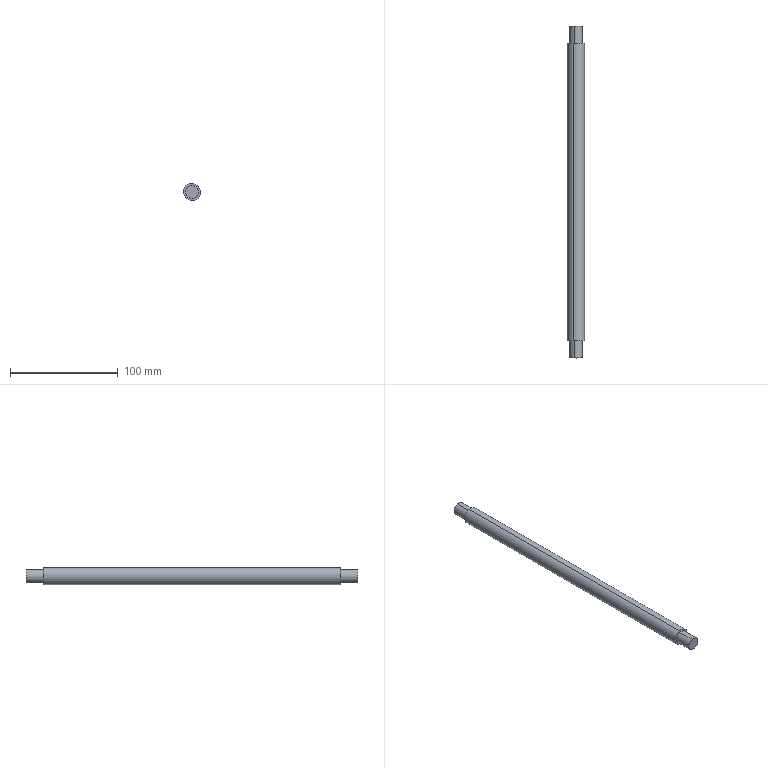Component | SolidWorks | AdjustmentRod-2 | 1 solid | 10 faces | box 16 x 308 x 16 mm | volume 59112 mm3 | cylinder 6 | plane 4 | commonest cylinder face diameters 12 x4 16 x2
build123d program:
from build123d import *


with BuildPart() as part:
    # Sketch1 → Revolve1 (revolve)
    with BuildSketch(Plane.XY, mode=Mode.PRIVATE) as revolve1_sk:
        Polygon((6, 154), (6, 138), (8, 138), (8, -138), (6, -138), (6, -154), (0, -154), (0, 154), align=None)
    revolve(revolve1_sk.sketch.rotate(Axis((0, 0, 0), (0, 1, 0)), 90), axis=Axis((0, 0, 0), (0, 1, 0)))


solid = part.part

# Placed as in the assembly
solid = solid.moved(Location((-155, 0, 0), (0, 0, 0)))
STEP:
#1=COLOUR_RGB('',0.7922,0.8196,0.9333);
#2=FILL_AREA_STYLE_COLOUR('',#1);
#3=FILL_AREA_STYLE('',(#2));
#4=SURFACE_STYLE_FILL_AREA(#3);
#5=SURFACE_SIDE_STYLE('',(#4));
#6=SURFACE_STYLE_USAGE(.BOTH.,#5);
#7=PRESENTATION_STYLE_ASSIGNMENT((#6));
#8=CARTESIAN_POINT('',(-6.035,6.063,-0.2263));
#9=VERTEX_POINT('',#8);
#10=CARTESIAN_POINT('',(-6.17,6.063,0.2263));
#11=VERTEX_POINT('',#10);
#12=CARTESIAN_POINT('',(-6.102,6.063,0.));
#13=DIRECTION('',(-0.,-1.,-0.));
#14=DIRECTION('',(0.2867,0.,-0.958));
#15=AXIS2_PLACEMENT_3D('',#12,#13,#14);
#16=CIRCLE('',#15,0.2362);
#17=EDGE_CURVE('',#9,#11,#16,.T.);
#18=ORIENTED_EDGE('',*,*,#17,.T.);
#19=CARTESIAN_POINT('',(-6.17,5.433,0.2263));
#20=VERTEX_POINT('',#19);
#21=CARTESIAN_POINT('',(-6.17,0.,0.2263));
#22=DIRECTION('',(-0.,-1.,-0.));
#23=VECTOR('',#22,39.37);
#24=LINE('',#21,#23);
#25=EDGE_CURVE('',#11,#20,#24,.T.);
#26=ORIENTED_EDGE('',*,*,#25,.T.);
#27=CARTESIAN_POINT('',(-6.035,5.433,-0.2263));
#28=VERTEX_POINT('',#27);
#29=CARTESIAN_POINT('',(-6.102,5.433,0.));
#30=DIRECTION('',(-0.,-1.,-0.));
#31=DIRECTION('',(0.2867,0.,-0.958));
#32=AXIS2_PLACEMENT_3D('',#29,#30,#31);
#33=CIRCLE('',#32,0.2362);
#34=EDGE_CURVE('',#28,#20,#33,.T.);
#35=ORIENTED_EDGE('',*,*,#34,.F.);
#36=CARTESIAN_POINT('',(-6.035,0.,-0.2263));
#37=DIRECTION('',(-0.,-1.,-0.));
#38=VECTOR('',#37,39.37);
#39=LINE('',#36,#38);
#40=EDGE_CURVE('',#9,#28,#39,.T.);
#41=ORIENTED_EDGE('',*,*,#40,.F.);
#42=EDGE_LOOP('',(#18,#26,#35,#41));
#43=FACE_OUTER_BOUND('',#42,.T.);
#44=CARTESIAN_POINT('',(-6.102,0.,-0.));
#45=DIRECTION('',(-0.,-1.,-0.));
#46=DIRECTION('',(0.2867,0.,-0.958));
#47=AXIS2_PLACEMENT_3D('',#44,#45,#46);
#48=CYLINDRICAL_SURFACE('',#47,0.2362);
#49=ADVANCED_FACE('',(#43),#48,.T.);
#50=CARTESIAN_POINT('',(-6.012,5.433,-0.3017));
#51=VERTEX_POINT('',#50);
#52=CARTESIAN_POINT('',(-6.193,5.433,0.3017));
#53=VERTEX_POINT('',#52);
#54=CARTESIAN_POINT('',(-6.102,5.433,0.));
#55=DIRECTION('',(-0.,-1.,-0.));
#56=DIRECTION('',(0.2867,0.,-0.958));
#57=AXIS2_PLACEMENT_3D('',#54,#55,#56);
#58=CIRCLE('',#57,0.315);
#59=EDGE_CURVE('',#51,#53,#58,.T.);
#60=ORIENTED_EDGE('',*,*,#59,.T.);
#61=CARTESIAN_POINT('',(-6.193,-5.433,0.3017));
#62=VERTEX_POINT('',#61);
#63=CARTESIAN_POINT('',(-6.193,0.,0.3017));
#64=DIRECTION('',(-0.,-1.,-0.));
#65=VECTOR('',#64,39.37);
#66=LINE('',#63,#65);
#67=EDGE_CURVE('',#53,#62,#66,.T.);
#68=ORIENTED_EDGE('',*,*,#67,.T.);
#69=CARTESIAN_POINT('',(-6.012,-5.433,-0.3017));
#70=VERTEX_POINT('',#69);
#71=CARTESIAN_POINT('',(-6.102,-5.433,-0.));
#72=DIRECTION('',(-0.,-1.,-0.));
#73=DIRECTION('',(0.2867,0.,-0.958));
#74=AXIS2_PLACEMENT_3D('',#71,#72,#73);
#75=CIRCLE('',#74,0.315);
#76=EDGE_CURVE('',#70,#62,#75,.T.);
#77=ORIENTED_EDGE('',*,*,#76,.F.);
#78=CARTESIAN_POINT('',(-6.012,0.,-0.3017));
#79=DIRECTION('',(-0.,-1.,-0.));
#80=VECTOR('',#79,39.37);
#81=LINE('',#78,#80);
#82=EDGE_CURVE('',#51,#70,#81,.T.);
#83=ORIENTED_EDGE('',*,*,#82,.F.);
#84=EDGE_LOOP('',(#60,#68,#77,#83));
#85=FACE_OUTER_BOUND('',#84,.T.);
#86=CARTESIAN_POINT('',(-6.102,0.,-0.));
#87=DIRECTION('',(-0.,-1.,-0.));
#88=DIRECTION('',(0.2867,0.,-0.958));
#89=AXIS2_PLACEMENT_3D('',#86,#87,#88);
#90=CYLINDRICAL_SURFACE('',#89,0.315);
#91=ADVANCED_FACE('',(#85),#90,.T.);
#92=CARTESIAN_POINT('',(-6.035,-5.433,-0.2263));
#93=VERTEX_POINT('',#92);
#94=CARTESIAN_POINT('',(-6.17,-5.433,0.2263));
#95=VERTEX_POINT('',#94);
#96=CARTESIAN_POINT('',(-6.102,-5.433,-0.));
#97=DIRECTION('',(-0.,-1.,-0.));
#98=DIRECTION('',(0.2867,0.,-0.958));
#99=AXIS2_PLACEMENT_3D('',#96,#97,#98);
#100=CIRCLE('',#99,0.2362);
#101=EDGE_CURVE('',#93,#95,#100,.T.);
#102=ORIENTED_EDGE('',*,*,#101,.T.);
#103=CARTESIAN_POINT('',(-6.17,-6.063,0.2263));
#104=VERTEX_POINT('',#103);
#105=CARTESIAN_POINT('',(-6.17,0.,0.2263));
#106=DIRECTION('',(-0.,-1.,-0.));
#107=VECTOR('',#106,39.37);
#108=LINE('',#105,#107);
#109=EDGE_CURVE('',#95,#104,#108,.T.);
#110=ORIENTED_EDGE('',*,*,#109,.T.);
#111=CARTESIAN_POINT('',(-6.035,-6.063,-0.2263));
#112=VERTEX_POINT('',#111);
#113=CARTESIAN_POINT('',(-6.102,-6.063,-0.));
#114=DIRECTION('',(-0.,-1.,-0.));
#115=DIRECTION('',(0.2867,0.,-0.958));
#116=AXIS2_PLACEMENT_3D('',#113,#114,#115);
#117=CIRCLE('',#116,0.2362);
#118=EDGE_CURVE('',#112,#104,#117,.T.);
#119=ORIENTED_EDGE('',*,*,#118,.F.);
#120=CARTESIAN_POINT('',(-6.035,0.,-0.2263));
#121=DIRECTION('',(-0.,-1.,-0.));
#122=VECTOR('',#121,39.37);
#123=LINE('',#120,#122);
#124=EDGE_CURVE('',#93,#112,#123,.T.);
#125=ORIENTED_EDGE('',*,*,#124,.F.);
#126=EDGE_LOOP('',(#102,#110,#119,#125));
#127=FACE_OUTER_BOUND('',#126,.T.);
#128=CARTESIAN_POINT('',(-6.102,0.,-0.));
#129=DIRECTION('',(-0.,-1.,-0.));
#130=DIRECTION('',(0.2867,0.,-0.958));
#131=AXIS2_PLACEMENT_3D('',#128,#129,#130);
#132=CYLINDRICAL_SURFACE('',#131,0.2362);
#133=ADVANCED_FACE('',(#127),#132,.T.);
#134=ORIENTED_EDGE('',*,*,#17,.F.);
#135=CARTESIAN_POINT('',(-6.102,6.063,0.));
#136=DIRECTION('',(-0.,-1.,-0.));
#137=DIRECTION('',(0.2867,0.,-0.958));
#138=AXIS2_PLACEMENT_3D('',#135,#136,#137);
#139=CIRCLE('',#138,0.2362);
#140=EDGE_CURVE('',#11,#9,#139,.T.);
#141=ORIENTED_EDGE('',*,*,#140,.F.);
#142=EDGE_LOOP('',(#134,#141));
#143=FACE_OUTER_BOUND('',#142,.T.);
#144=CARTESIAN_POINT('',(-5.876,6.063,0.06773));
#145=DIRECTION('',(0.,1.,0.));
#146=DIRECTION('',(-0.2867,-0.,0.958));
#147=AXIS2_PLACEMENT_3D('',#144,#145,#146);
#148=PLANE('',#147);
#149=ADVANCED_FACE('',(#143),#148,.T.);
#150=ORIENTED_EDGE('',*,*,#118,.T.);
#151=CARTESIAN_POINT('',(-6.102,-6.063,-0.));
#152=DIRECTION('',(-0.,-1.,-0.));
#153=DIRECTION('',(0.2867,0.,-0.958));
#154=AXIS2_PLACEMENT_3D('',#151,#152,#153);
#155=CIRCLE('',#154,0.2362);
#156=EDGE_CURVE('',#104,#112,#155,.T.);
#157=ORIENTED_EDGE('',*,*,#156,.T.);
#158=EDGE_LOOP('',(#150,#157));
#159=FACE_OUTER_BOUND('',#158,.T.);
#160=CARTESIAN_POINT('',(-6.102,-6.063,-0.));
#161=DIRECTION('',(-0.,-1.,-0.));
#162=DIRECTION('',(0.2867,0.,-0.958));
#163=AXIS2_PLACEMENT_3D('',#160,#161,#162);
#164=PLANE('',#163);
#165=ADVANCED_FACE('',(#159),#164,.T.);
#166=ORIENTED_EDGE('',*,*,#109,.F.);
#167=CARTESIAN_POINT('',(-6.102,-5.433,-0.));
#168=DIRECTION('',(-0.,-1.,-0.));
#169=DIRECTION('',(0.2867,0.,-0.958));
#170=AXIS2_PLACEMENT_3D('',#167,#168,#169);
#171=CIRCLE('',#170,0.2362);
#172=EDGE_CURVE('',#95,#93,#171,.T.);
#173=ORIENTED_EDGE('',*,*,#172,.T.);
#174=ORIENTED_EDGE('',*,*,#124,.T.);
#175=ORIENTED_EDGE('',*,*,#156,.F.);
#176=EDGE_LOOP('',(#166,#173,#174,#175));
#177=FACE_OUTER_BOUND('',#176,.T.);
#178=CARTESIAN_POINT('',(-6.102,0.,-0.));
#179=DIRECTION('',(-0.,-1.,-0.));
#180=DIRECTION('',(0.2867,0.,-0.958));
#181=AXIS2_PLACEMENT_3D('',#178,#179,#180);
#182=CYLINDRICAL_SURFACE('',#181,0.2362);
#183=ADVANCED_FACE('',(#177),#182,.T.);
#184=ORIENTED_EDGE('',*,*,#76,.T.);
#185=CARTESIAN_POINT('',(-6.102,-5.433,-0.));
#186=DIRECTION('',(-0.,-1.,-0.));
#187=DIRECTION('',(0.2867,0.,-0.958));
#188=AXIS2_PLACEMENT_3D('',#185,#186,#187);
#189=CIRCLE('',#188,0.315);
#190=EDGE_CURVE('',#62,#70,#189,.T.);
#191=ORIENTED_EDGE('',*,*,#190,.T.);
#192=EDGE_LOOP('',(#184,#191));
#193=FACE_OUTER_BOUND('',#192,.T.);
#194=ORIENTED_EDGE('',*,*,#101,.F.);
#195=ORIENTED_EDGE('',*,*,#172,.F.);
#196=EDGE_LOOP('',(#194,#195));
#197=FACE_BOUND('',#196,.T.);
#198=CARTESIAN_POINT('',(-5.876,-5.433,0.06773));
#199=DIRECTION('',(-0.,-1.,-0.));
#200=DIRECTION('',(0.2867,0.,-0.958));
#201=AXIS2_PLACEMENT_3D('',#198,#199,#200);
#202=PLANE('',#201);
#203=ADVANCED_FACE('',(#193,#197),#202,.T.);
#204=ORIENTED_EDGE('',*,*,#67,.F.);
#205=CARTESIAN_POINT('',(-6.102,5.433,0.));
#206=DIRECTION('',(-0.,-1.,-0.));
#207=DIRECTION('',(0.2867,0.,-0.958));
#208=AXIS2_PLACEMENT_3D('',#205,#206,#207);
#209=CIRCLE('',#208,0.315);
#210=EDGE_CURVE('',#53,#51,#209,.T.);
#211=ORIENTED_EDGE('',*,*,#210,.T.);
#212=ORIENTED_EDGE('',*,*,#82,.T.);
#213=ORIENTED_EDGE('',*,*,#190,.F.);
#214=EDGE_LOOP('',(#204,#211,#212,#213));
#215=FACE_OUTER_BOUND('',#214,.T.);
#216=CARTESIAN_POINT('',(-6.102,0.,-0.));
#217=DIRECTION('',(-0.,-1.,-0.));
#218=DIRECTION('',(0.2867,0.,-0.958));
#219=AXIS2_PLACEMENT_3D('',#216,#217,#218);
#220=CYLINDRICAL_SURFACE('',#219,0.315);
#221=ADVANCED_FACE('',(#215),#220,.T.);
#222=ORIENTED_EDGE('',*,*,#34,.T.);
#223=CARTESIAN_POINT('',(-6.102,5.433,0.));
#224=DIRECTION('',(-0.,-1.,-0.));
#225=DIRECTION('',(0.2867,0.,-0.958));
#226=AXIS2_PLACEMENT_3D('',#223,#224,#225);
#227=CIRCLE('',#226,0.2362);
#228=EDGE_CURVE('',#20,#28,#227,.T.);
#229=ORIENTED_EDGE('',*,*,#228,.T.);
#230=EDGE_LOOP('',(#222,#229));
#231=FACE_BOUND('',#230,.T.);
#232=ORIENTED_EDGE('',*,*,#59,.F.);
#233=ORIENTED_EDGE('',*,*,#210,.F.);
#234=EDGE_LOOP('',(#232,#233));
#235=FACE_OUTER_BOUND('',#234,.T.);
#236=CARTESIAN_POINT('',(-5.876,5.433,0.06773));
#237=DIRECTION('',(0.,1.,0.));
#238=DIRECTION('',(-0.2867,-0.,0.958));
#239=AXIS2_PLACEMENT_3D('',#236,#237,#238);
#240=PLANE('',#239);
#241=ADVANCED_FACE('',(#231,#235),#240,.T.);
#242=ORIENTED_EDGE('',*,*,#25,.F.);
#243=ORIENTED_EDGE('',*,*,#140,.T.);
#244=ORIENTED_EDGE('',*,*,#40,.T.);
#245=ORIENTED_EDGE('',*,*,#228,.F.);
#246=EDGE_LOOP('',(#242,#243,#244,#245));
#247=FACE_OUTER_BOUND('',#246,.T.);
#248=CARTESIAN_POINT('',(-6.102,0.,-0.));
#249=DIRECTION('',(-0.,-1.,-0.));
#250=DIRECTION('',(0.2867,0.,-0.958));
#251=AXIS2_PLACEMENT_3D('',#248,#249,#250);
#252=CYLINDRICAL_SURFACE('',#251,0.2362);
#253=ADVANCED_FACE('',(#247),#252,.T.);
#254=CLOSED_SHELL('',(#49,#91,#133,#149,#165,#183,#203,#221,#241,#253));
#255=MANIFOLD_SOLID_BREP('',#254);
#256=STYLED_ITEM('',(#7),#255);
#257=(LENGTH_UNIT()NAMED_UNIT(*)SI_UNIT($,.METRE.));
#258=LENGTH_MEASURE_WITH_UNIT(LENGTH_MEASURE(0.0254),#257);
#259=DIMENSIONAL_EXPONENTS(1.,0.,0.,0.,0.,0.,0.);
#260=(CONVERSION_BASED_UNIT('',#258)LENGTH_UNIT()NAMED_UNIT(#259));
#261=UNCERTAINTY_MEASURE_WITH_UNIT(LENGTH_MEASURE(0.00001),#260,'','');
#262=(NAMED_UNIT(*)PLANE_ANGLE_UNIT()SI_UNIT($,.RADIAN.));
#263=(NAMED_UNIT(*)SI_UNIT($,.STERADIAN.)SOLID_ANGLE_UNIT());
#264=(GEOMETRIC_REPRESENTATION_CONTEXT(3)GLOBAL_UNCERTAINTY_ASSIGNED_CONTEXT((#261))GLOBAL_UNIT_ASSIGNED_CONTEXT((#260,#262,#263))REPRESENTATION_CONTEXT('',''));
#265=MECHANICAL_DESIGN_GEOMETRIC_PRESENTATION_REPRESENTATION('',(#256),#264);
#266=CARTESIAN_POINT('',(0.,0.,0.));
#267=DIRECTION('',(0.,0.,1.));
#268=DIRECTION('',(1.,0.,0.));
#269=AXIS2_PLACEMENT_3D('',#266,#267,#268);
#270=(LENGTH_UNIT()NAMED_UNIT(*)SI_UNIT($,.METRE.));
#271=LENGTH_MEASURE_WITH_UNIT(LENGTH_MEASURE(0.0254),#270);
#272=DIMENSIONAL_EXPONENTS(1.,0.,0.,0.,0.,0.,0.);
#273=(CONVERSION_BASED_UNIT('',#271)LENGTH_UNIT()NAMED_UNIT(#272));
#274=UNCERTAINTY_MEASURE_WITH_UNIT(LENGTH_MEASURE(0.00001),#273,'','');
#275=(NAMED_UNIT(*)PLANE_ANGLE_UNIT()SI_UNIT($,.RADIAN.));
#276=(NAMED_UNIT(*)SI_UNIT($,.STERADIAN.)SOLID_ANGLE_UNIT());
#277=(GEOMETRIC_REPRESENTATION_CONTEXT(3)GLOBAL_UNCERTAINTY_ASSIGNED_CONTEXT((#274))GLOBAL_UNIT_ASSIGNED_CONTEXT((#273,#275,#276))REPRESENTATION_CONTEXT('',''));
#278=ADVANCED_BREP_SHAPE_REPRESENTATION('',(#255,#269),#277);
#279=PRESENTATION_LAYER_ASSIGNMENT('','',(#256));